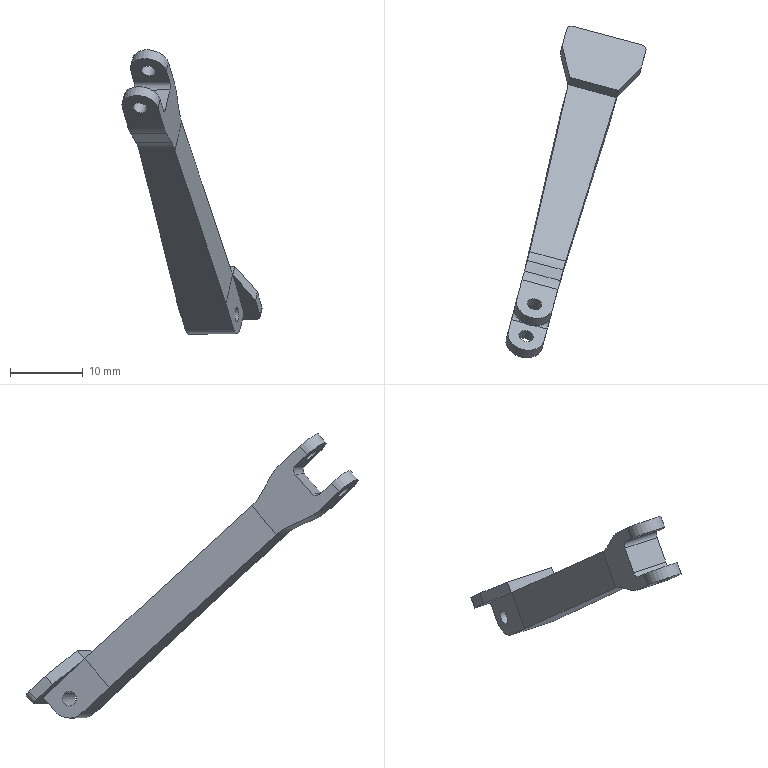Component | NX | CONNECTING_ROD_2 | 1 solid | 38 faces | volume 1734 mm3 | plane 24 | cylinder 14 | commonest cylinder face diameters 12.7 x4 1.587 x4 2 x3 5.08 x2 5.292 x1